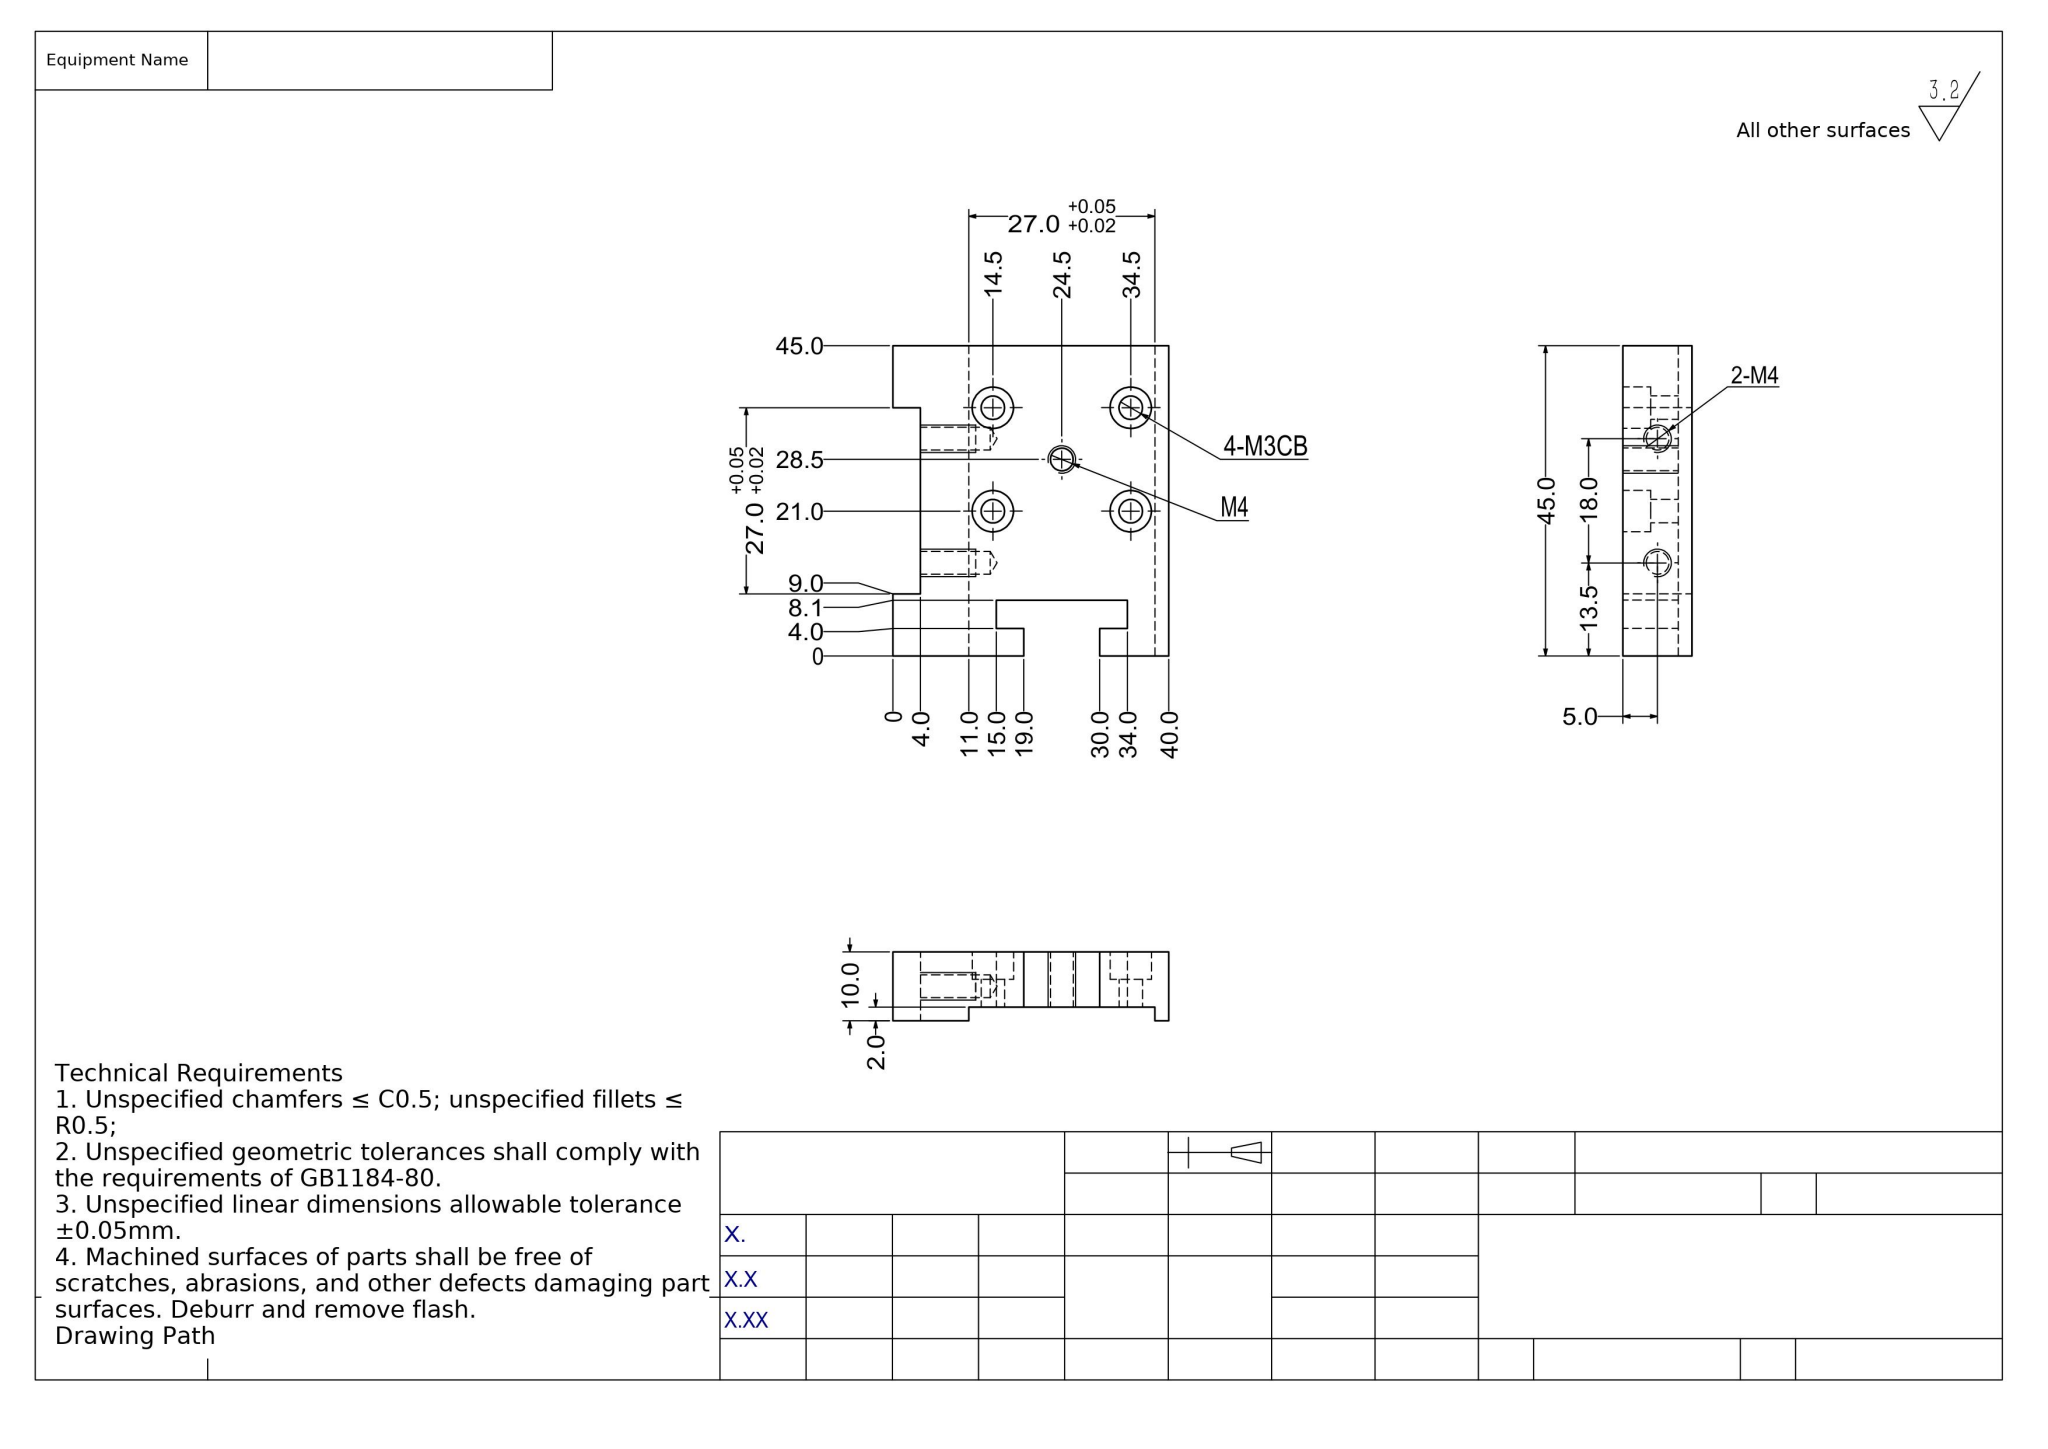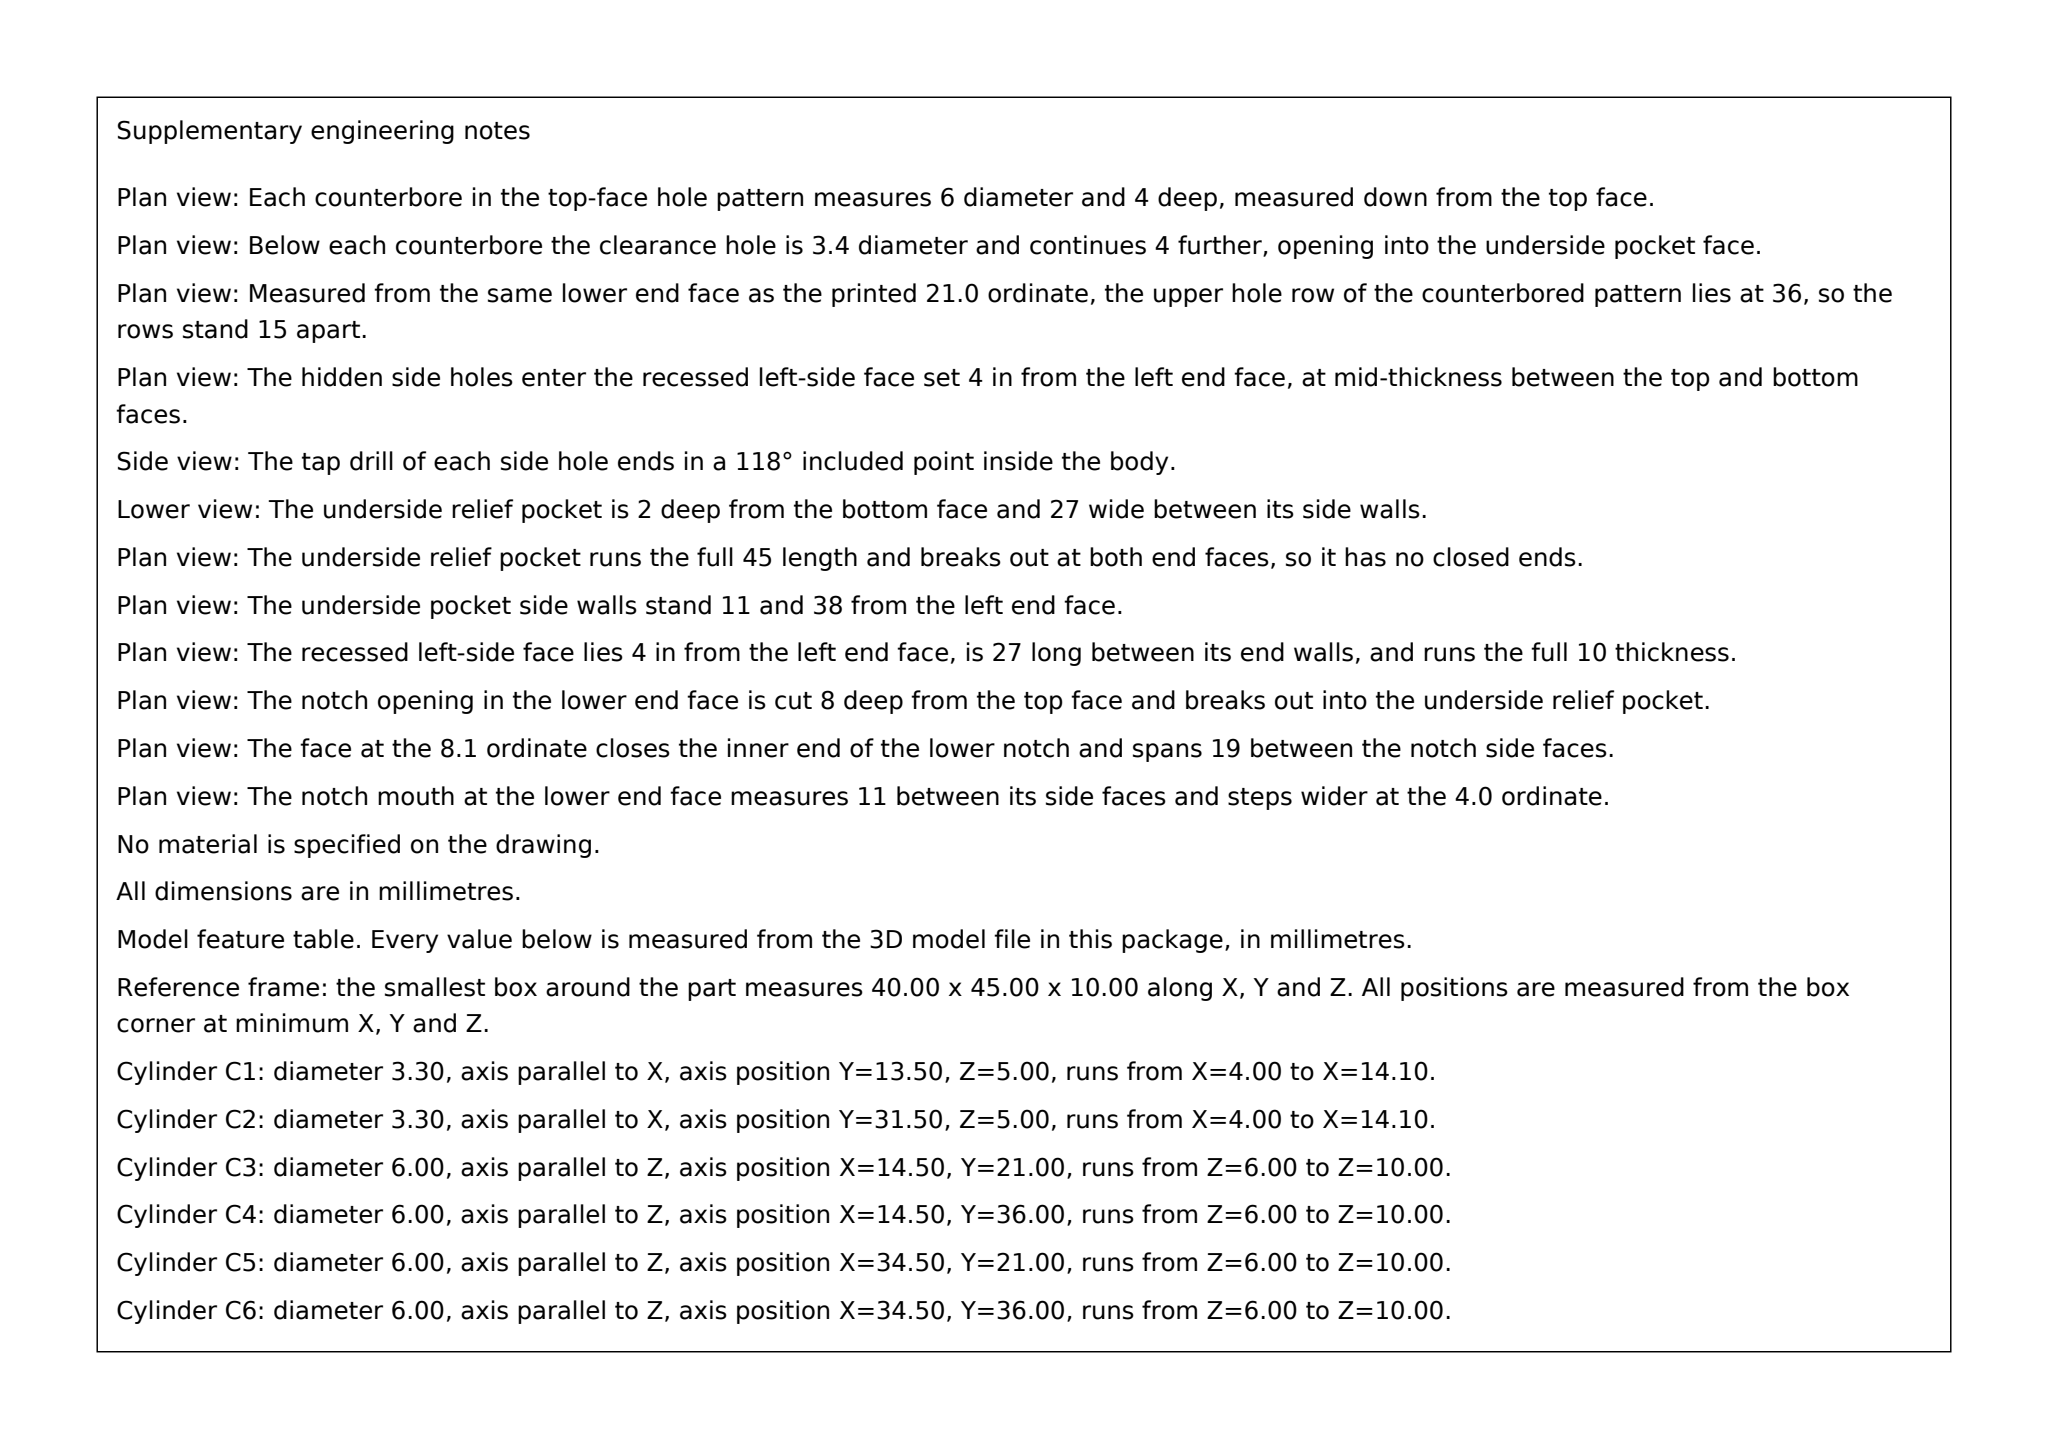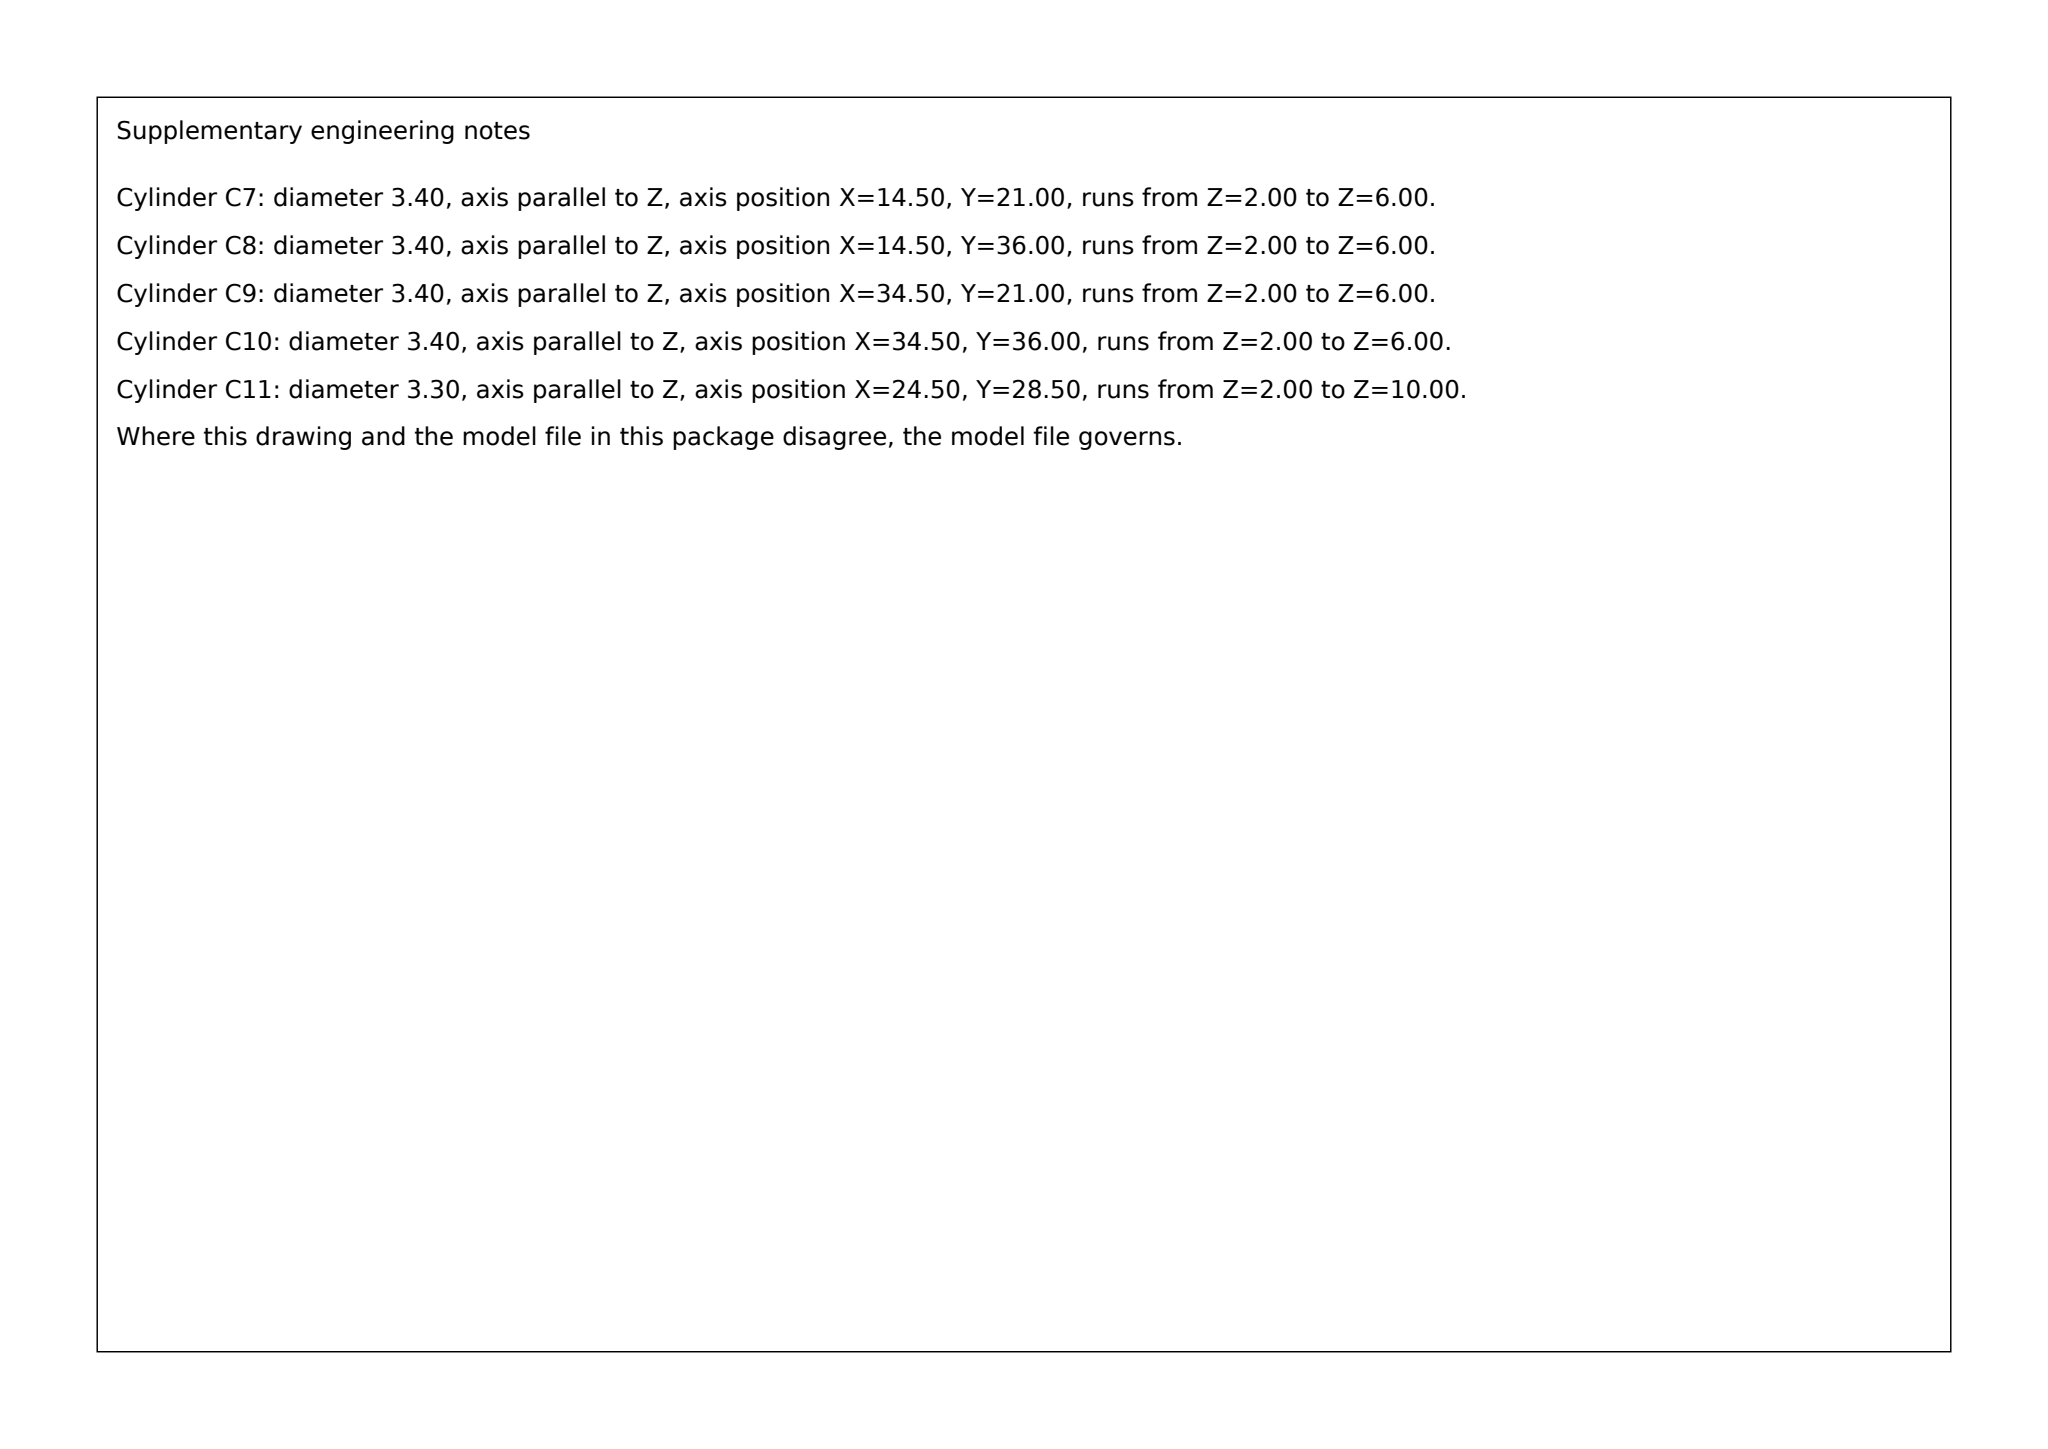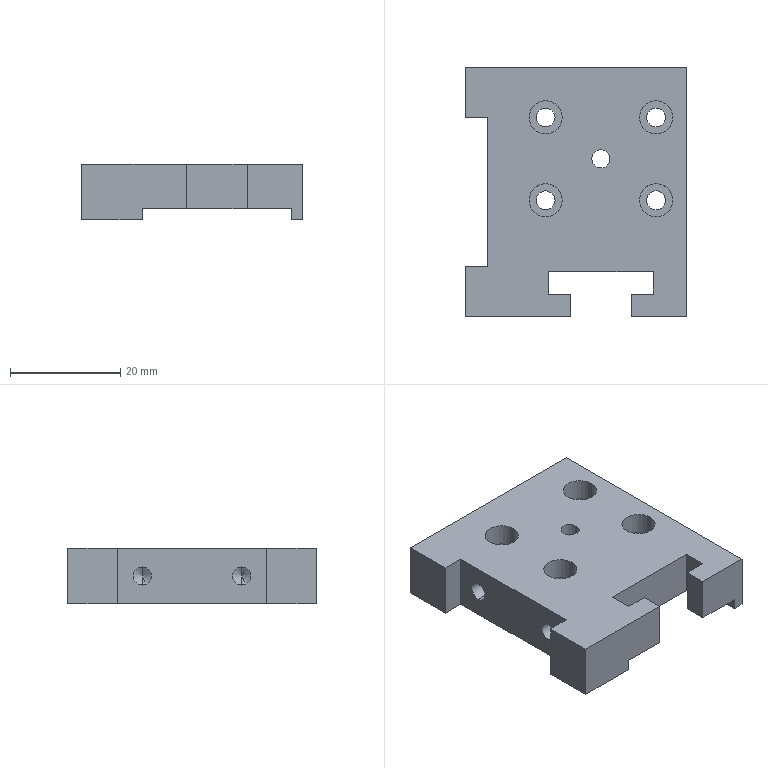Part | SolidWorks | mm | 1 solid | 52 faces | box 40 x 45 x 10 mm | volume 12670 mm3 | plane 26 | cylinder 22 | cone 4 | commonest cylinder face diameters 6 x8 3.4 x8 3.3 x6
Drawing notes:
4-M3CB: C'BORE Ø6.0, 4.0 DEEP FROM TOP (10.0) FACE | from the solid: cyl dia 6.0 axis z len 4.0 at (14.5/34.5, 21.0/36.0); z planes 10.0 & 6.0
4-M3CB C'BORE FLOOR AT Z=6.0, i.e. 4.0 BELOW 10.0 FACE | from the solid: axis_planes z=6.0 (4 faces), z=10.0 top face
4-M3CB: Ø3.4 THRU (4.0 DEEP, Z6.0 TO Z2.0 FACE) | from the solid: cyl dia 3.4 axis z len 4.0 at 4 positions; z planes 6.0 and 2.0
M4 AT 24.5,28.5: TAP DRILL Ø3.3 DP 8.0 FROM TOP (10.0) FACE | from the solid: cyl dia 3.3 axis z pos(24.5,28.5) len 8.0; cone 118° ref dia 3.3
2-M4 SIDE HOLES: THD DP 10.1 FROM LH END FACE | from the solid: cyl dia 3.3 axis x at y13.5 & y31.5, z5.0, len 10.1
2-M4 SIDE: TAP DRILL Ø3.3 DP 10.1 FROM LH END FACE (X=0) | from the solid: cyl dia 3.3 axis x len 10.1; x planes 0.0 start, hidden detail to x=11
FRONT VIEW: ADD ORDINATE 38.0 AT BOTTOM RELIEF END FACE | from the solid: axis_planes x=38.0 (1), bbox X=40.0
UNDERSIDE RELIEF (FLOOR Z=2.0): X 19.0 TO 38.0, 2.0 LAND TO X40.0 | from the solid: x planes 19.0,38.0,40.0; z plane 2.0; bbox 40x45x10
build123d program:
from build123d import *

# Parameters (mm, degrees)
SKETCH1_W             = 40
SKETCH1_H             = 45
BOSS_EXTRUDE1_DEPTH   = 10
SKETCH11_R            = 1.7
CUT_EXTRUDE5_DEPTH    = 62.033
SKETCH12_R            = 3
CUT_EXTRUDE6_DEPTH    = 4
SKETCH16_W            = 11
SKETCH16_H            = 19.5
CUT_EXTRUDE9_DEPTH    = 62.033
SKETCH17_W            = 19
SKETCH17_H            = 4.1
CUT_EXTRUDE10_DEPTH   = 62.033
M4_TAPPED_HOLE1_D     = 3.3
SKETCH13_W            = 27
SKETCH13_H            = 45
CUT_EXTRUDE11_DEPTH   = 2
SKETCH31_W            = 10
SKETCH31_H            = 27
CUT_EXTRUDE12_DEPTH   = 4
M4_TAPPED_HOLE2_D     = 3.3
M4_TAPPED_HOLE2_DEPTH = 10.1
M4_TAPPED_HOLE2_TIP   = 0.9914


with BuildPart() as part:
    # Sketch1 → Boss-Extrude1 (new body)
    with BuildSketch(Plane.XY):
        with Locations((20, 22.5)):
            Rectangle(SKETCH1_W, SKETCH1_H)
    extrude(amount=BOSS_EXTRUDE1_DEPTH)

    # Sketch11 → Cut-Extrude5 (cut, through all)
    with BuildSketch(Plane(origin=(0, 0, 0), x_dir=(-1, 0, 0), z_dir=(0, 0, -1))):
        with Locations((-34.5, 36)):
            Circle(SKETCH11_R)
        with Locations((-34.5, 21)):
            Circle(SKETCH11_R)
        with Locations((-14.5, 21)):
            Circle(SKETCH11_R)
        with Locations((-14.5, 36)):
            Circle(SKETCH11_R)
    extrude(amount=-CUT_EXTRUDE5_DEPTH, mode=Mode.SUBTRACT)

    # Sketch12 → Cut-Extrude6 (cut)
    with BuildSketch(Plane.XY.offset(10)):
        with Locations((14.5, 36)):
            Circle(SKETCH12_R)
        with Locations((34.5, 36)):
            Circle(SKETCH12_R)
        with Locations((34.5, 21)):
            Circle(SKETCH12_R)
        with Locations((14.5, 21)):
            Circle(SKETCH12_R)
    extrude(amount=-CUT_EXTRUDE6_DEPTH, mode=Mode.SUBTRACT)

    # Sketch16 → Cut-Extrude9 (cut, through all)
    with BuildSketch(Plane.XY.offset(10)):
        with Locations((24.5, -5.75)):
            Rectangle(SKETCH16_W, SKETCH16_H)
    extrude(amount=-CUT_EXTRUDE9_DEPTH, mode=Mode.SUBTRACT)

    # Sketch17 → Cut-Extrude10 (cut, through all)
    with BuildSketch(Plane.XY.offset(10)):
        with Locations((24.5, 6.05)):
            Rectangle(SKETCH17_W, SKETCH17_H)
    extrude(amount=-CUT_EXTRUDE10_DEPTH, mode=Mode.SUBTRACT)

    # M4 Tapped Hole1 (through all)
    with Locations(Plane.XY.offset(10)):
        with Locations((24.5, 28.5)):
            Hole(M4_TAPPED_HOLE1_D / 2)

    # Sketch13 → Cut-Extrude11 (cut)
    with BuildSketch(Plane(origin=(0, 0, 0), x_dir=(-1, 0, 0), z_dir=(0, 0, -1))):
        with Locations((-24.5, 22.5)):
            Rectangle(SKETCH13_W, SKETCH13_H)
    extrude(amount=-CUT_EXTRUDE11_DEPTH, mode=Mode.SUBTRACT)

    # Sketch31 → Cut-Extrude12 (cut)
    with BuildSketch(Plane.ZY):
        with Locations((5, 22.5)):
            Rectangle(SKETCH31_W, SKETCH31_H)
    extrude(amount=-CUT_EXTRUDE12_DEPTH, mode=Mode.SUBTRACT)

    # M4 Tapped Hole2
    with Locations(Plane.ZY.offset(-4)):
        with Locations((5, 31.5), (5, 13.5)):
            Hole(M4_TAPPED_HOLE2_D / 2, depth=M4_TAPPED_HOLE2_DEPTH)
            with Locations((0, 0, -(M4_TAPPED_HOLE2_DEPTH + M4_TAPPED_HOLE2_TIP / 2))):  # 118° drill point
                Cone(0, M4_TAPPED_HOLE2_D / 2, M4_TAPPED_HOLE2_TIP, mode=Mode.SUBTRACT)


solid = part.part